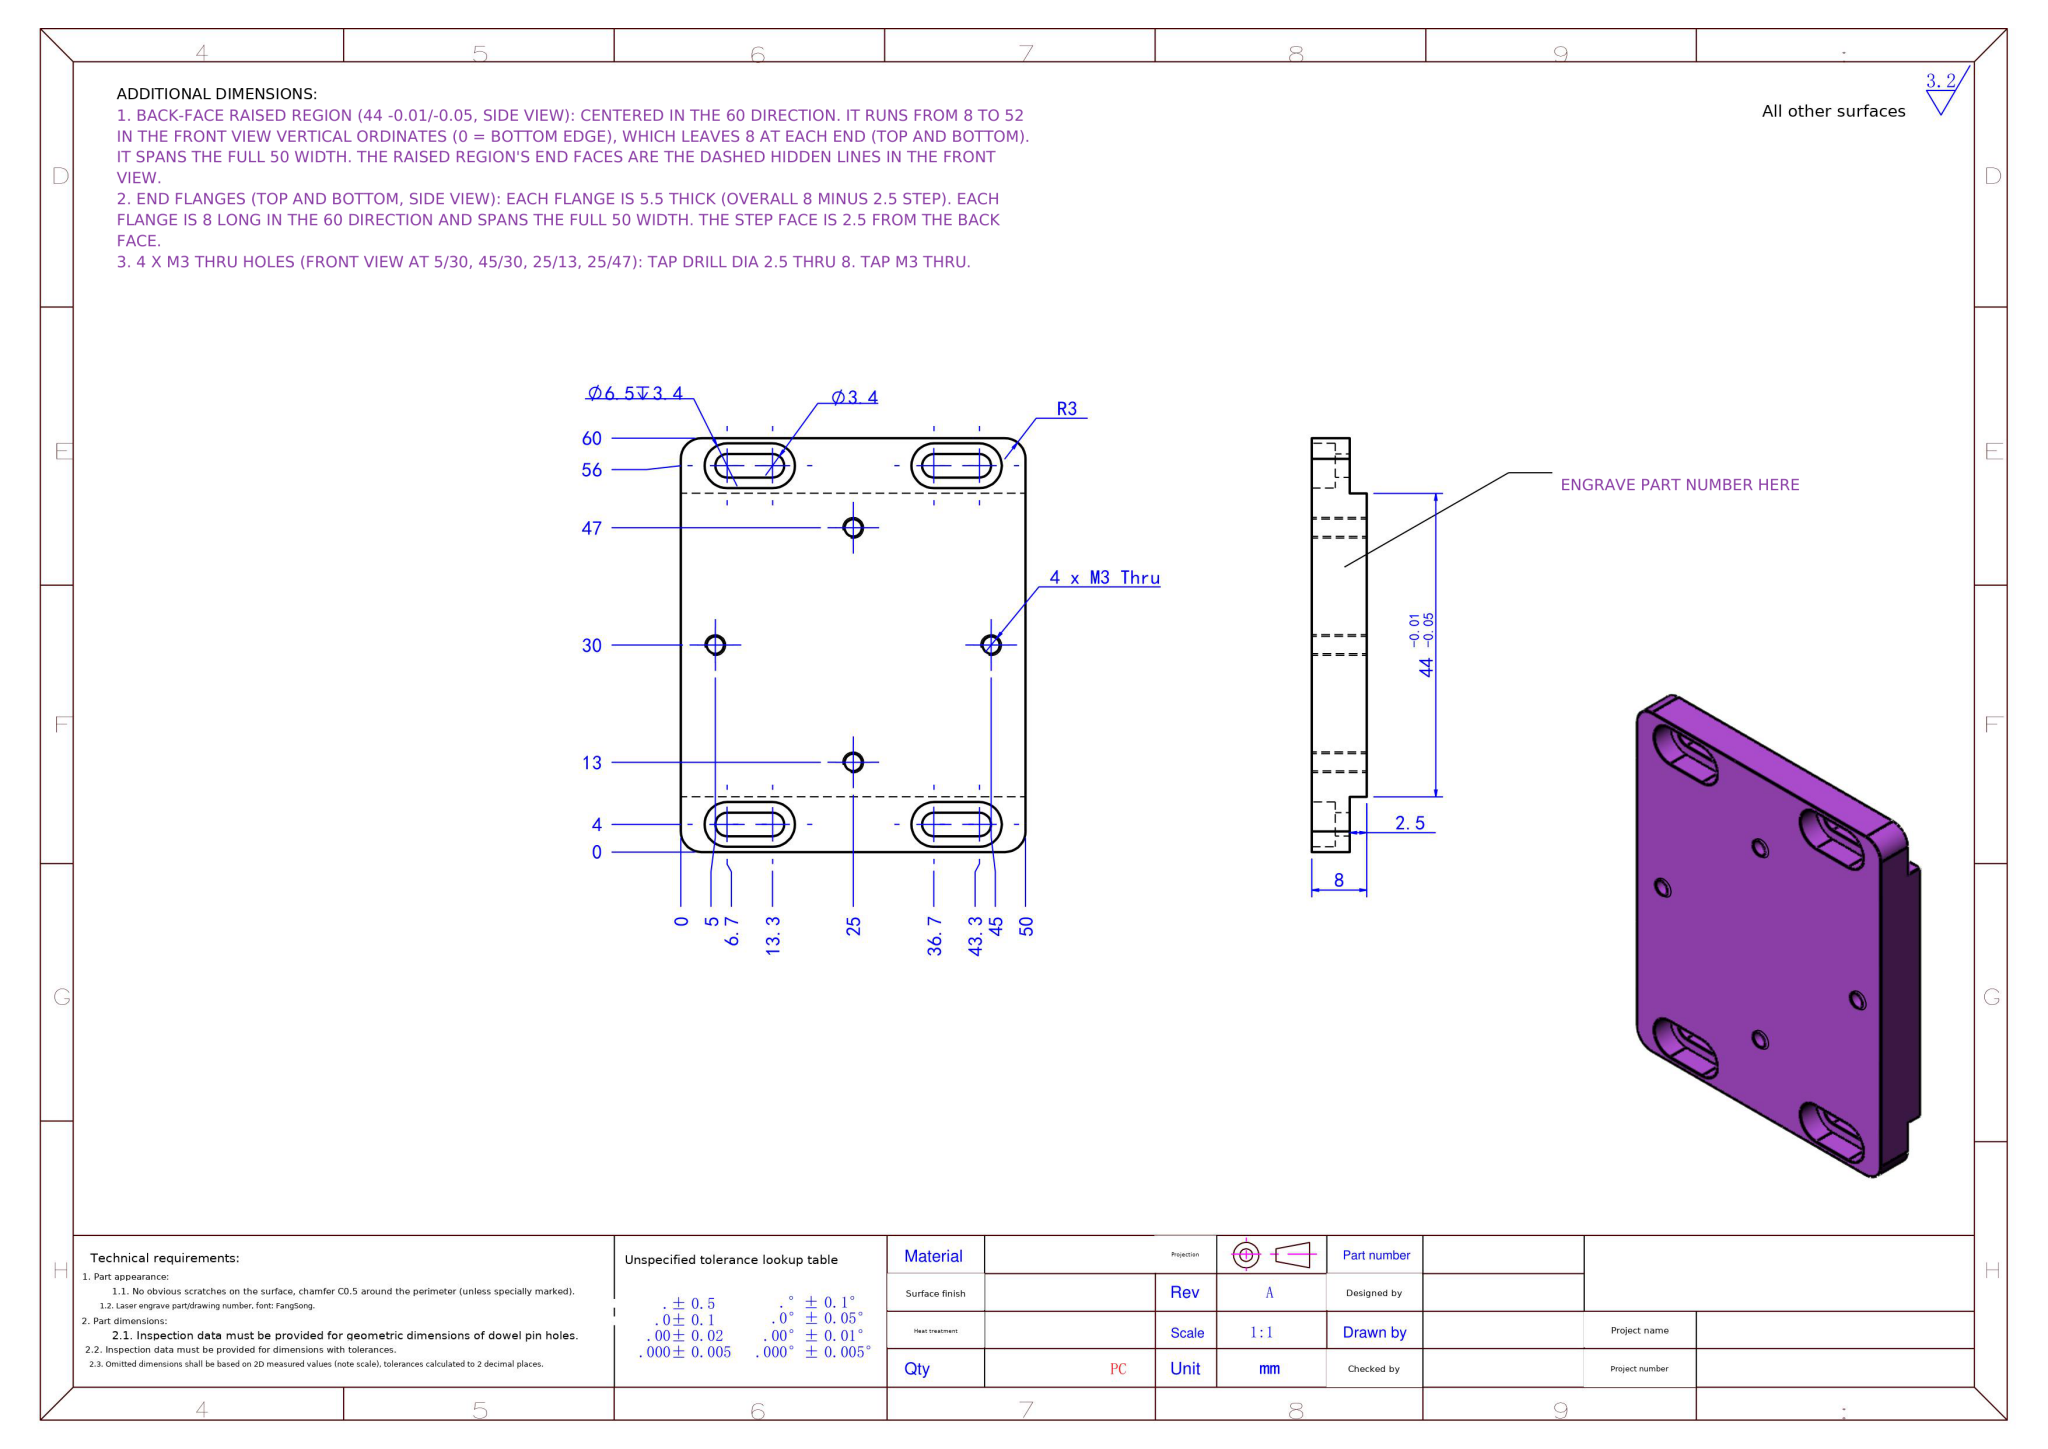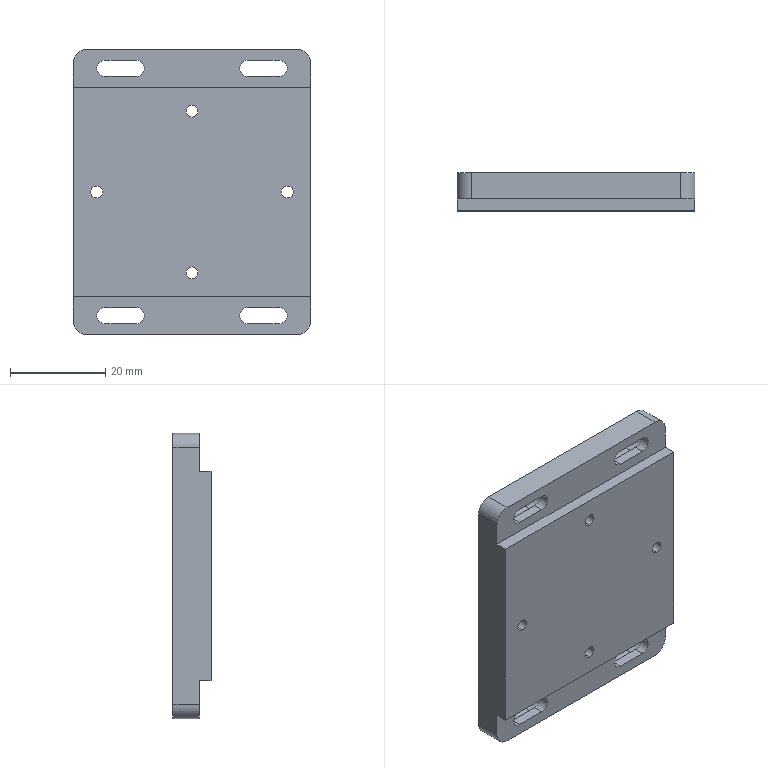Part | NX | mm | 1 solid | 58 faces | box 50 x 8 x 60 mm | volume 20501 mm3 | plane 30 | cylinder 28 | commonest cylinder face diameters 2.5 x8 3.4 x8 6.5 x8 6 x4